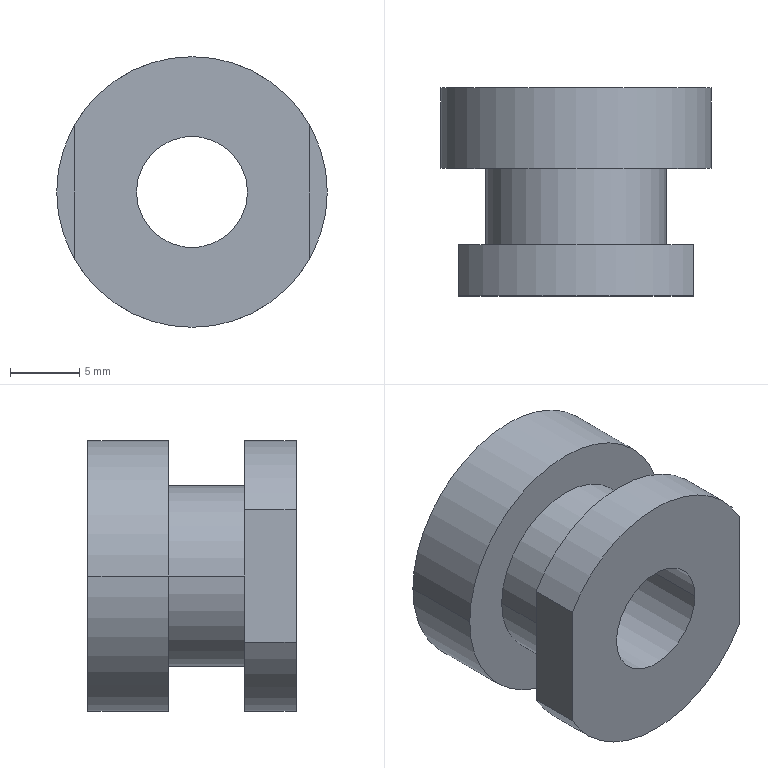Component | SolidWorks | HandlingMechanism-2_A070-1 | 1 solid | 14 faces | box 19.5 x 15 x 19.5 mm | volume 2753 mm3 | cylinder 8 | plane 6 | commonest cylinder face diameters 19.5 x4 8 x2 13 x2
build123d program:
from build123d import *

# Parameters (mm, degrees)
SKETCH1_R           = 9.75
BOSS_EXTRUDE1_DEPTH = 15
SKETCH2_W           = 3.25
SKETCH2_H           = 5.5
SKETCH3_W           = 1.25
SKETCH3_H           = 3.7
CUT_EXTRUDE1_DEPTH  = 7.5
M8_TAPPED_HOLE1_D   = 8


with BuildPart() as part:
    # Sketch1 → Boss-Extrude1 (new body)
    with BuildSketch(Plane.XY):
        Circle(SKETCH1_R)
    extrude(amount=BOSS_EXTRUDE1_DEPTH)

    # Sketch2 → Cut-Revolve1 (revolve, cut)
    with BuildSketch(Plane(origin=(0, 0, 0), x_dir=(1, 0, 0), z_dir=(0, 1, 0)), mode=Mode.PRIVATE) as cut_revolve1_sk:
        with Locations((-8.125, -8.55)):
            Rectangle(SKETCH2_W, SKETCH2_H)
    revolve(cut_revolve1_sk.sketch.rotate(Axis((0, 0, 15), (0, 0, -1)), 180), axis=Axis((0, 0, 15), (0, 0, -1)), mode=Mode.SUBTRACT)

    # Sketch3 → Cut-Extrude1 (cut, symmetric)
    with BuildSketch(Plane(origin=(0, 0, 0), x_dir=(1, 0, 0), z_dir=(0, 1, 0))):
        with Locations((-9.125, -13.15)):
            Rectangle(SKETCH3_W, SKETCH3_H)
        with Locations((9.125, -13.15)):
            Rectangle(SKETCH3_W, SKETCH3_H)
    extrude(amount=CUT_EXTRUDE1_DEPTH, both=True, mode=Mode.SUBTRACT)

    # M8 Tapped Hole1 (through all)
    with Locations(Plane.XY.offset(15)):
        with Locations((0, 0)):
            Hole(M8_TAPPED_HOLE1_D / 2)


solid = part.part

# Placed as in the assembly
solid = solid.moved(Location((25.881, 139.5, 151), (90, 0, 0)))
STEP:
#1=CARTESIAN_POINT('',(1.176,5.492,5.945));
#2=VERTEX_POINT('',#1);
#3=CARTESIAN_POINT('',(0.8614,5.492,5.945));
#4=VERTEX_POINT('',#3);
#5=CARTESIAN_POINT('',(1.019,5.492,5.945));
#6=DIRECTION('',(0.,-1.,-0.));
#7=DIRECTION('',(-1.,-0.,-0.));
#8=AXIS2_PLACEMENT_3D('',#5,#6,#7);
#9=CIRCLE('',#8,0.1575);
#10=EDGE_CURVE('',#2,#4,#9,.T.);
#11=ORIENTED_EDGE('',*,*,#10,.F.);
#12=CARTESIAN_POINT('',(1.176,4.902,5.945));
#13=VERTEX_POINT('',#12);
#14=CARTESIAN_POINT('',(1.176,4.902,5.945));
#15=DIRECTION('',(0.,-1.,-0.));
#16=VECTOR('',#15,39.37);
#17=LINE('',#14,#16);
#18=EDGE_CURVE('',#2,#13,#17,.T.);
#19=ORIENTED_EDGE('',*,*,#18,.T.);
#20=CARTESIAN_POINT('',(0.8614,4.902,5.945));
#21=VERTEX_POINT('',#20);
#22=CARTESIAN_POINT('',(1.019,4.902,5.945));
#23=DIRECTION('',(0.,-1.,-0.));
#24=DIRECTION('',(-1.,-0.,-0.));
#25=AXIS2_PLACEMENT_3D('',#22,#23,#24);
#26=CIRCLE('',#25,0.1575);
#27=EDGE_CURVE('',#13,#21,#26,.T.);
#28=ORIENTED_EDGE('',*,*,#27,.T.);
#29=CARTESIAN_POINT('',(0.8614,4.902,5.945));
#30=DIRECTION('',(0.,-1.,-0.));
#31=VECTOR('',#30,39.37);
#32=LINE('',#29,#31);
#33=EDGE_CURVE('',#4,#21,#32,.T.);
#34=ORIENTED_EDGE('',*,*,#33,.F.);
#35=EDGE_LOOP('',(#11,#19,#28,#34));
#36=FACE_OUTER_BOUND('',#35,.T.);
#37=CARTESIAN_POINT('',(1.019,4.902,5.945));
#38=DIRECTION('',(0.,-1.,-0.));
#39=DIRECTION('',(-1.,-0.,-0.));
#40=AXIS2_PLACEMENT_3D('',#37,#38,#39);
#41=CYLINDRICAL_SURFACE('',#40,0.1575);
#42=ADVANCED_FACE('',(#36),#41,.F.);
#43=CARTESIAN_POINT('',(0.6351,5.264,5.945));
#44=VERTEX_POINT('',#43);
#45=CARTESIAN_POINT('',(1.403,5.264,5.945));
#46=VERTEX_POINT('',#45);
#47=CARTESIAN_POINT('',(1.019,5.264,5.945));
#48=DIRECTION('',(0.,-1.,-0.));
#49=DIRECTION('',(-1.,-0.,-0.));
#50=AXIS2_PLACEMENT_3D('',#47,#48,#49);
#51=CIRCLE('',#50,0.3839);
#52=EDGE_CURVE('',#44,#46,#51,.T.);
#53=ORIENTED_EDGE('',*,*,#52,.F.);
#54=CARTESIAN_POINT('',(0.6351,5.492,5.945));
#55=VERTEX_POINT('',#54);
#56=CARTESIAN_POINT('',(0.6351,4.902,5.945));
#57=DIRECTION('',(-0.,1.,0.));
#58=VECTOR('',#57,39.37);
#59=LINE('',#56,#58);
#60=EDGE_CURVE('',#44,#55,#59,.T.);
#61=ORIENTED_EDGE('',*,*,#60,.T.);
#62=CARTESIAN_POINT('',(1.403,5.492,5.945));
#63=VERTEX_POINT('',#62);
#64=CARTESIAN_POINT('',(1.019,5.492,5.945));
#65=DIRECTION('',(0.,-1.,-0.));
#66=DIRECTION('',(-1.,-0.,-0.));
#67=AXIS2_PLACEMENT_3D('',#64,#65,#66);
#68=CIRCLE('',#67,0.3839);
#69=EDGE_CURVE('',#55,#63,#68,.T.);
#70=ORIENTED_EDGE('',*,*,#69,.T.);
#71=CARTESIAN_POINT('',(1.403,4.902,5.945));
#72=DIRECTION('',(-0.,1.,0.));
#73=VECTOR('',#72,39.37);
#74=LINE('',#71,#73);
#75=EDGE_CURVE('',#46,#63,#74,.T.);
#76=ORIENTED_EDGE('',*,*,#75,.F.);
#77=EDGE_LOOP('',(#53,#61,#70,#76));
#78=FACE_OUTER_BOUND('',#77,.T.);
#79=CARTESIAN_POINT('',(1.019,4.902,5.945));
#80=DIRECTION('',(-0.,1.,0.));
#81=DIRECTION('',(1.,0.,0.));
#82=AXIS2_PLACEMENT_3D('',#79,#80,#81);
#83=CYLINDRICAL_SURFACE('',#82,0.3839);
#84=ADVANCED_FACE('',(#78),#83,.T.);
#85=CARTESIAN_POINT('',(0.763,5.264,5.945));
#86=VERTEX_POINT('',#85);
#87=CARTESIAN_POINT('',(1.275,5.264,5.945));
#88=VERTEX_POINT('',#87);
#89=CARTESIAN_POINT('',(1.019,5.264,5.945));
#90=DIRECTION('',(0.,-1.,-0.));
#91=DIRECTION('',(-1.,-0.,-0.));
#92=AXIS2_PLACEMENT_3D('',#89,#90,#91);
#93=CIRCLE('',#92,0.2559);
#94=EDGE_CURVE('',#86,#88,#93,.T.);
#95=ORIENTED_EDGE('',*,*,#94,.T.);
#96=CARTESIAN_POINT('',(1.275,5.047,5.945));
#97=VERTEX_POINT('',#96);
#98=CARTESIAN_POINT('',(1.275,4.902,5.945));
#99=DIRECTION('',(0.,-1.,-0.));
#100=VECTOR('',#99,39.37);
#101=LINE('',#98,#100);
#102=EDGE_CURVE('',#88,#97,#101,.T.);
#103=ORIENTED_EDGE('',*,*,#102,.T.);
#104=CARTESIAN_POINT('',(0.763,5.047,5.945));
#105=VERTEX_POINT('',#104);
#106=CARTESIAN_POINT('',(1.019,5.047,5.945));
#107=DIRECTION('',(0.,-1.,-0.));
#108=DIRECTION('',(-1.,-0.,-0.));
#109=AXIS2_PLACEMENT_3D('',#106,#107,#108);
#110=CIRCLE('',#109,0.2559);
#111=EDGE_CURVE('',#105,#97,#110,.T.);
#112=ORIENTED_EDGE('',*,*,#111,.F.);
#113=CARTESIAN_POINT('',(0.763,4.902,5.945));
#114=DIRECTION('',(0.,-1.,-0.));
#115=VECTOR('',#114,39.37);
#116=LINE('',#113,#115);
#117=EDGE_CURVE('',#86,#105,#116,.T.);
#118=ORIENTED_EDGE('',*,*,#117,.F.);
#119=EDGE_LOOP('',(#95,#103,#112,#118));
#120=FACE_OUTER_BOUND('',#119,.T.);
#121=CARTESIAN_POINT('',(1.019,4.902,5.945));
#122=DIRECTION('',(0.,-1.,-0.));
#123=DIRECTION('',(-1.,-0.,-0.));
#124=AXIS2_PLACEMENT_3D('',#121,#122,#123);
#125=CYLINDRICAL_SURFACE('',#124,0.2559);
#126=ADVANCED_FACE('',(#120),#125,.T.);
#127=CARTESIAN_POINT('',(0.6843,4.902,5.757));
#128=VERTEX_POINT('',#127);
#129=CARTESIAN_POINT('',(1.354,4.902,5.757));
#130=VERTEX_POINT('',#129);
#131=CARTESIAN_POINT('',(1.019,4.902,5.945));
#132=DIRECTION('',(0.,-1.,-0.));
#133=DIRECTION('',(-1.,-0.,-0.));
#134=AXIS2_PLACEMENT_3D('',#131,#132,#133);
#135=CIRCLE('',#134,0.3839);
#136=EDGE_CURVE('',#128,#130,#135,.T.);
#137=ORIENTED_EDGE('',*,*,#136,.F.);
#138=CARTESIAN_POINT('',(0.6843,5.047,5.757));
#139=VERTEX_POINT('',#138);
#140=CARTESIAN_POINT('',(0.6843,4.902,5.757));
#141=DIRECTION('',(-0.,1.,0.));
#142=VECTOR('',#141,39.37);
#143=LINE('',#140,#142);
#144=EDGE_CURVE('',#128,#139,#143,.T.);
#145=ORIENTED_EDGE('',*,*,#144,.T.);
#146=CARTESIAN_POINT('',(1.354,5.047,5.757));
#147=VERTEX_POINT('',#146);
#148=CARTESIAN_POINT('',(1.019,5.047,5.945));
#149=DIRECTION('',(0.,-1.,-0.));
#150=DIRECTION('',(-1.,-0.,-0.));
#151=AXIS2_PLACEMENT_3D('',#148,#149,#150);
#152=CIRCLE('',#151,0.3839);
#153=EDGE_CURVE('',#139,#147,#152,.T.);
#154=ORIENTED_EDGE('',*,*,#153,.T.);
#155=CARTESIAN_POINT('',(1.354,4.902,5.757));
#156=DIRECTION('',(0.,-1.,-0.));
#157=VECTOR('',#156,39.37);
#158=LINE('',#155,#157);
#159=EDGE_CURVE('',#147,#130,#158,.T.);
#160=ORIENTED_EDGE('',*,*,#159,.T.);
#161=EDGE_LOOP('',(#137,#145,#154,#160));
#162=FACE_OUTER_BOUND('',#161,.T.);
#163=CARTESIAN_POINT('',(1.019,4.902,5.945));
#164=DIRECTION('',(-0.,1.,0.));
#165=DIRECTION('',(1.,0.,0.));
#166=AXIS2_PLACEMENT_3D('',#163,#164,#165);
#167=CYLINDRICAL_SURFACE('',#166,0.3839);
#168=ADVANCED_FACE('',(#162),#167,.T.);
#169=CARTESIAN_POINT('',(1.354,5.047,6.133));
#170=VERTEX_POINT('',#169);
#171=CARTESIAN_POINT('',(0.6843,5.047,6.133));
#172=VERTEX_POINT('',#171);
#173=CARTESIAN_POINT('',(1.019,5.047,5.945));
#174=DIRECTION('',(0.,-1.,-0.));
#175=DIRECTION('',(-1.,-0.,-0.));
#176=AXIS2_PLACEMENT_3D('',#173,#174,#175);
#177=CIRCLE('',#176,0.3839);
#178=EDGE_CURVE('',#170,#172,#177,.T.);
#179=ORIENTED_EDGE('',*,*,#178,.T.);
#180=CARTESIAN_POINT('',(0.6843,4.902,6.133));
#181=VERTEX_POINT('',#180);
#182=CARTESIAN_POINT('',(0.6843,4.902,6.133));
#183=DIRECTION('',(0.,-1.,-0.));
#184=VECTOR('',#183,39.37);
#185=LINE('',#182,#184);
#186=EDGE_CURVE('',#172,#181,#185,.T.);
#187=ORIENTED_EDGE('',*,*,#186,.T.);
#188=CARTESIAN_POINT('',(1.354,4.902,6.133));
#189=VERTEX_POINT('',#188);
#190=CARTESIAN_POINT('',(1.019,4.902,5.945));
#191=DIRECTION('',(0.,-1.,-0.));
#192=DIRECTION('',(-1.,-0.,-0.));
#193=AXIS2_PLACEMENT_3D('',#190,#191,#192);
#194=CIRCLE('',#193,0.3839);
#195=EDGE_CURVE('',#189,#181,#194,.T.);
#196=ORIENTED_EDGE('',*,*,#195,.F.);
#197=CARTESIAN_POINT('',(1.354,4.902,6.133));
#198=DIRECTION('',(-0.,1.,0.));
#199=VECTOR('',#198,39.37);
#200=LINE('',#197,#199);
#201=EDGE_CURVE('',#189,#170,#200,.T.);
#202=ORIENTED_EDGE('',*,*,#201,.T.);
#203=EDGE_LOOP('',(#179,#187,#196,#202));
#204=FACE_OUTER_BOUND('',#203,.T.);
#205=CARTESIAN_POINT('',(1.019,4.902,5.945));
#206=DIRECTION('',(-0.,1.,0.));
#207=DIRECTION('',(1.,0.,0.));
#208=AXIS2_PLACEMENT_3D('',#205,#206,#207);
#209=CYLINDRICAL_SURFACE('',#208,0.3839);
#210=ADVANCED_FACE('',(#204),#209,.T.);
#211=CARTESIAN_POINT('',(1.019,4.902,5.945));
#212=DIRECTION('',(0.,-1.,-0.));
#213=DIRECTION('',(-1.,-0.,-0.));
#214=AXIS2_PLACEMENT_3D('',#211,#212,#213);
#215=CIRCLE('',#214,0.1575);
#216=EDGE_CURVE('',#21,#13,#215,.T.);
#217=ORIENTED_EDGE('',*,*,#216,.F.);
#218=ORIENTED_EDGE('',*,*,#27,.F.);
#219=EDGE_LOOP('',(#217,#218));
#220=FACE_BOUND('',#219,.T.);
#221=CARTESIAN_POINT('',(0.6843,4.902,6.24));
#222=DIRECTION('',(0.,0.,-1.));
#223=VECTOR('',#222,39.37);
#224=LINE('',#221,#223);
#225=EDGE_CURVE('',#181,#128,#224,.T.);
#226=ORIENTED_EDGE('',*,*,#225,.T.);
#227=ORIENTED_EDGE('',*,*,#136,.T.);
#228=CARTESIAN_POINT('',(1.354,4.902,6.24));
#229=DIRECTION('',(0.,0.,-1.));
#230=VECTOR('',#229,39.37);
#231=LINE('',#228,#230);
#232=EDGE_CURVE('',#189,#130,#231,.T.);
#233=ORIENTED_EDGE('',*,*,#232,.F.);
#234=ORIENTED_EDGE('',*,*,#195,.T.);
#235=EDGE_LOOP('',(#226,#227,#233,#234));
#236=FACE_OUTER_BOUND('',#235,.T.);
#237=CARTESIAN_POINT('',(1.019,4.902,5.945));
#238=DIRECTION('',(0.,-1.,-0.));
#239=DIRECTION('',(-1.,-0.,-0.));
#240=AXIS2_PLACEMENT_3D('',#237,#238,#239);
#241=PLANE('',#240);
#242=ADVANCED_FACE('',(#220,#236),#241,.T.);
#243=CARTESIAN_POINT('',(0.6843,5.047,5.945));
#244=DIRECTION('',(0.,0.,-1.));
#245=VECTOR('',#244,39.37);
#246=LINE('',#243,#245);
#247=EDGE_CURVE('',#172,#139,#246,.T.);
#248=ORIENTED_EDGE('',*,*,#247,.F.);
#249=ORIENTED_EDGE('',*,*,#178,.F.);
#250=CARTESIAN_POINT('',(1.354,5.047,5.945));
#251=DIRECTION('',(-0.,-0.,1.));
#252=VECTOR('',#251,39.37);
#253=LINE('',#250,#252);
#254=EDGE_CURVE('',#147,#170,#253,.T.);
#255=ORIENTED_EDGE('',*,*,#254,.F.);
#256=ORIENTED_EDGE('',*,*,#153,.F.);
#257=EDGE_LOOP('',(#248,#249,#255,#256));
#258=FACE_OUTER_BOUND('',#257,.T.);
#259=ORIENTED_EDGE('',*,*,#111,.T.);
#260=CARTESIAN_POINT('',(1.019,5.047,5.945));
#261=DIRECTION('',(0.,-1.,-0.));
#262=DIRECTION('',(-1.,-0.,-0.));
#263=AXIS2_PLACEMENT_3D('',#260,#261,#262);
#264=CIRCLE('',#263,0.2559);
#265=EDGE_CURVE('',#97,#105,#264,.T.);
#266=ORIENTED_EDGE('',*,*,#265,.T.);
#267=EDGE_LOOP('',(#259,#266));
#268=FACE_BOUND('',#267,.T.);
#269=CARTESIAN_POINT('',(1.403,5.047,5.945));
#270=DIRECTION('',(-0.,1.,0.));
#271=DIRECTION('',(1.,0.,0.));
#272=AXIS2_PLACEMENT_3D('',#269,#270,#271);
#273=PLANE('',#272);
#274=ADVANCED_FACE('',(#258,#268),#273,.T.);
#275=ORIENTED_EDGE('',*,*,#102,.F.);
#276=CARTESIAN_POINT('',(1.019,5.264,5.945));
#277=DIRECTION('',(0.,-1.,-0.));
#278=DIRECTION('',(-1.,-0.,-0.));
#279=AXIS2_PLACEMENT_3D('',#276,#277,#278);
#280=CIRCLE('',#279,0.2559);
#281=EDGE_CURVE('',#88,#86,#280,.T.);
#282=ORIENTED_EDGE('',*,*,#281,.T.);
#283=ORIENTED_EDGE('',*,*,#117,.T.);
#284=ORIENTED_EDGE('',*,*,#265,.F.);
#285=EDGE_LOOP('',(#275,#282,#283,#284));
#286=FACE_OUTER_BOUND('',#285,.T.);
#287=CARTESIAN_POINT('',(1.019,4.902,5.945));
#288=DIRECTION('',(0.,-1.,-0.));
#289=DIRECTION('',(-1.,-0.,-0.));
#290=AXIS2_PLACEMENT_3D('',#287,#288,#289);
#291=CYLINDRICAL_SURFACE('',#290,0.2559);
#292=ADVANCED_FACE('',(#286),#291,.T.);
#293=CARTESIAN_POINT('',(1.019,5.264,5.945));
#294=DIRECTION('',(0.,-1.,-0.));
#295=DIRECTION('',(-1.,-0.,-0.));
#296=AXIS2_PLACEMENT_3D('',#293,#294,#295);
#297=CIRCLE('',#296,0.3839);
#298=EDGE_CURVE('',#46,#44,#297,.T.);
#299=ORIENTED_EDGE('',*,*,#298,.T.);
#300=ORIENTED_EDGE('',*,*,#52,.T.);
#301=EDGE_LOOP('',(#299,#300));
#302=FACE_OUTER_BOUND('',#301,.T.);
#303=ORIENTED_EDGE('',*,*,#94,.F.);
#304=ORIENTED_EDGE('',*,*,#281,.F.);
#305=EDGE_LOOP('',(#303,#304));
#306=FACE_BOUND('',#305,.T.);
#307=CARTESIAN_POINT('',(1.403,5.264,5.945));
#308=DIRECTION('',(0.,-1.,-0.));
#309=DIRECTION('',(-1.,-0.,-0.));
#310=AXIS2_PLACEMENT_3D('',#307,#308,#309);
#311=PLANE('',#310);
#312=ADVANCED_FACE('',(#302,#306),#311,.T.);
#313=CARTESIAN_POINT('',(1.019,5.492,5.945));
#314=DIRECTION('',(0.,-1.,-0.));
#315=DIRECTION('',(-1.,-0.,-0.));
#316=AXIS2_PLACEMENT_3D('',#313,#314,#315);
#317=CIRCLE('',#316,0.1575);
#318=EDGE_CURVE('',#4,#2,#317,.T.);
#319=ORIENTED_EDGE('',*,*,#318,.T.);
#320=ORIENTED_EDGE('',*,*,#10,.T.);
#321=EDGE_LOOP('',(#319,#320));
#322=FACE_BOUND('',#321,.T.);
#323=CARTESIAN_POINT('',(1.019,5.492,5.945));
#324=DIRECTION('',(0.,-1.,-0.));
#325=DIRECTION('',(-1.,-0.,-0.));
#326=AXIS2_PLACEMENT_3D('',#323,#324,#325);
#327=CIRCLE('',#326,0.3839);
#328=EDGE_CURVE('',#63,#55,#327,.T.);
#329=ORIENTED_EDGE('',*,*,#328,.F.);
#330=ORIENTED_EDGE('',*,*,#69,.F.);
#331=EDGE_LOOP('',(#329,#330));
#332=FACE_OUTER_BOUND('',#331,.T.);
#333=CARTESIAN_POINT('',(1.019,5.492,5.945));
#334=DIRECTION('',(0.,-1.,-0.));
#335=DIRECTION('',(-1.,-0.,-0.));
#336=AXIS2_PLACEMENT_3D('',#333,#334,#335);
#337=PLANE('',#336);
#338=ADVANCED_FACE('',(#322,#332),#337,.F.);
#339=ORIENTED_EDGE('',*,*,#60,.F.);
#340=ORIENTED_EDGE('',*,*,#298,.F.);
#341=ORIENTED_EDGE('',*,*,#75,.T.);
#342=ORIENTED_EDGE('',*,*,#328,.T.);
#343=EDGE_LOOP('',(#339,#340,#341,#342));
#344=FACE_OUTER_BOUND('',#343,.T.);
#345=CARTESIAN_POINT('',(1.019,4.902,5.945));
#346=DIRECTION('',(-0.,1.,0.));
#347=DIRECTION('',(1.,0.,0.));
#348=AXIS2_PLACEMENT_3D('',#345,#346,#347);
#349=CYLINDRICAL_SURFACE('',#348,0.3839);
#350=ADVANCED_FACE('',(#344),#349,.T.);
#351=ORIENTED_EDGE('',*,*,#232,.T.);
#352=ORIENTED_EDGE('',*,*,#159,.F.);
#353=ORIENTED_EDGE('',*,*,#254,.T.);
#354=ORIENTED_EDGE('',*,*,#201,.F.);
#355=EDGE_LOOP('',(#351,#352,#353,#354));
#356=FACE_OUTER_BOUND('',#355,.T.);
#357=CARTESIAN_POINT('',(1.354,5.047,6.24));
#358=DIRECTION('',(-1.,-0.,-0.));
#359=DIRECTION('',(-0.,1.,0.));
#360=AXIS2_PLACEMENT_3D('',#357,#358,#359);
#361=PLANE('',#360);
#362=ADVANCED_FACE('',(#356),#361,.F.);
#363=ORIENTED_EDGE('',*,*,#225,.F.);
#364=ORIENTED_EDGE('',*,*,#186,.F.);
#365=ORIENTED_EDGE('',*,*,#247,.T.);
#366=ORIENTED_EDGE('',*,*,#144,.F.);
#367=EDGE_LOOP('',(#363,#364,#365,#366));
#368=FACE_OUTER_BOUND('',#367,.T.);
#369=CARTESIAN_POINT('',(0.6843,5.047,6.24));
#370=DIRECTION('',(1.,0.,0.));
#371=DIRECTION('',(0.,-1.,-0.));
#372=AXIS2_PLACEMENT_3D('',#369,#370,#371);
#373=PLANE('',#372);
#374=ADVANCED_FACE('',(#368),#373,.F.);
#375=ORIENTED_EDGE('',*,*,#18,.F.);
#376=ORIENTED_EDGE('',*,*,#318,.F.);
#377=ORIENTED_EDGE('',*,*,#33,.T.);
#378=ORIENTED_EDGE('',*,*,#216,.T.);
#379=EDGE_LOOP('',(#375,#376,#377,#378));
#380=FACE_OUTER_BOUND('',#379,.T.);
#381=CARTESIAN_POINT('',(1.019,4.902,5.945));
#382=DIRECTION('',(0.,-1.,-0.));
#383=DIRECTION('',(-1.,-0.,-0.));
#384=AXIS2_PLACEMENT_3D('',#381,#382,#383);
#385=CYLINDRICAL_SURFACE('',#384,0.1575);
#386=ADVANCED_FACE('',(#380),#385,.F.);
#387=CLOSED_SHELL('',(#42,#84,#126,#168,#210,#242,#274,#292,#312,#338,#350,#362,#374,#386));
#388=MANIFOLD_SOLID_BREP('',#387);
#389=CARTESIAN_POINT('',(0.,0.,0.));
#390=DIRECTION('',(0.,0.,1.));
#391=DIRECTION('',(1.,0.,0.));
#392=AXIS2_PLACEMENT_3D('',#389,#390,#391);
#393=(LENGTH_UNIT()NAMED_UNIT(*)SI_UNIT($,.METRE.));
#394=LENGTH_MEASURE_WITH_UNIT(LENGTH_MEASURE(0.0254),#393);
#395=DIMENSIONAL_EXPONENTS(1.,0.,0.,0.,0.,0.,0.);
#396=(CONVERSION_BASED_UNIT('',#394)LENGTH_UNIT()NAMED_UNIT(#395));
#397=UNCERTAINTY_MEASURE_WITH_UNIT(LENGTH_MEASURE(0.00001),#396,'','');
#398=(NAMED_UNIT(*)PLANE_ANGLE_UNIT()SI_UNIT($,.RADIAN.));
#399=(NAMED_UNIT(*)SI_UNIT($,.STERADIAN.)SOLID_ANGLE_UNIT());
#400=(GEOMETRIC_REPRESENTATION_CONTEXT(3)GLOBAL_UNCERTAINTY_ASSIGNED_CONTEXT((#397))GLOBAL_UNIT_ASSIGNED_CONTEXT((#396,#398,#399))REPRESENTATION_CONTEXT('',''));
#401=ADVANCED_BREP_SHAPE_REPRESENTATION('',(#388,#392),#400);
#402=COLOUR_RGB('',0.7922,0.8196,0.9333);
#403=FILL_AREA_STYLE_COLOUR('',#402);
#404=FILL_AREA_STYLE('',(#403));
#405=SURFACE_STYLE_FILL_AREA(#404);
#406=SURFACE_SIDE_STYLE('',(#405));
#407=SURFACE_STYLE_USAGE(.BOTH.,#406);
#408=PRESENTATION_STYLE_ASSIGNMENT((#407));
#409=STYLED_ITEM('',(#408),#388);
#410=PRESENTATION_LAYER_ASSIGNMENT('','',(#409));
#411=(LENGTH_UNIT()NAMED_UNIT(*)SI_UNIT($,.METRE.));
#412=LENGTH_MEASURE_WITH_UNIT(LENGTH_MEASURE(0.0254),#411);
#413=DIMENSIONAL_EXPONENTS(1.,0.,0.,0.,0.,0.,0.);
#414=(CONVERSION_BASED_UNIT('',#412)LENGTH_UNIT()NAMED_UNIT(#413));
#415=UNCERTAINTY_MEASURE_WITH_UNIT(LENGTH_MEASURE(0.00001),#414,'','');
#416=(NAMED_UNIT(*)PLANE_ANGLE_UNIT()SI_UNIT($,.RADIAN.));
#417=(NAMED_UNIT(*)SI_UNIT($,.STERADIAN.)SOLID_ANGLE_UNIT());
#418=(GEOMETRIC_REPRESENTATION_CONTEXT(3)GLOBAL_UNCERTAINTY_ASSIGNED_CONTEXT((#415))GLOBAL_UNIT_ASSIGNED_CONTEXT((#414,#416,#417))REPRESENTATION_CONTEXT('',''));
#419=MECHANICAL_DESIGN_GEOMETRIC_PRESENTATION_REPRESENTATION('',(#409),#418);